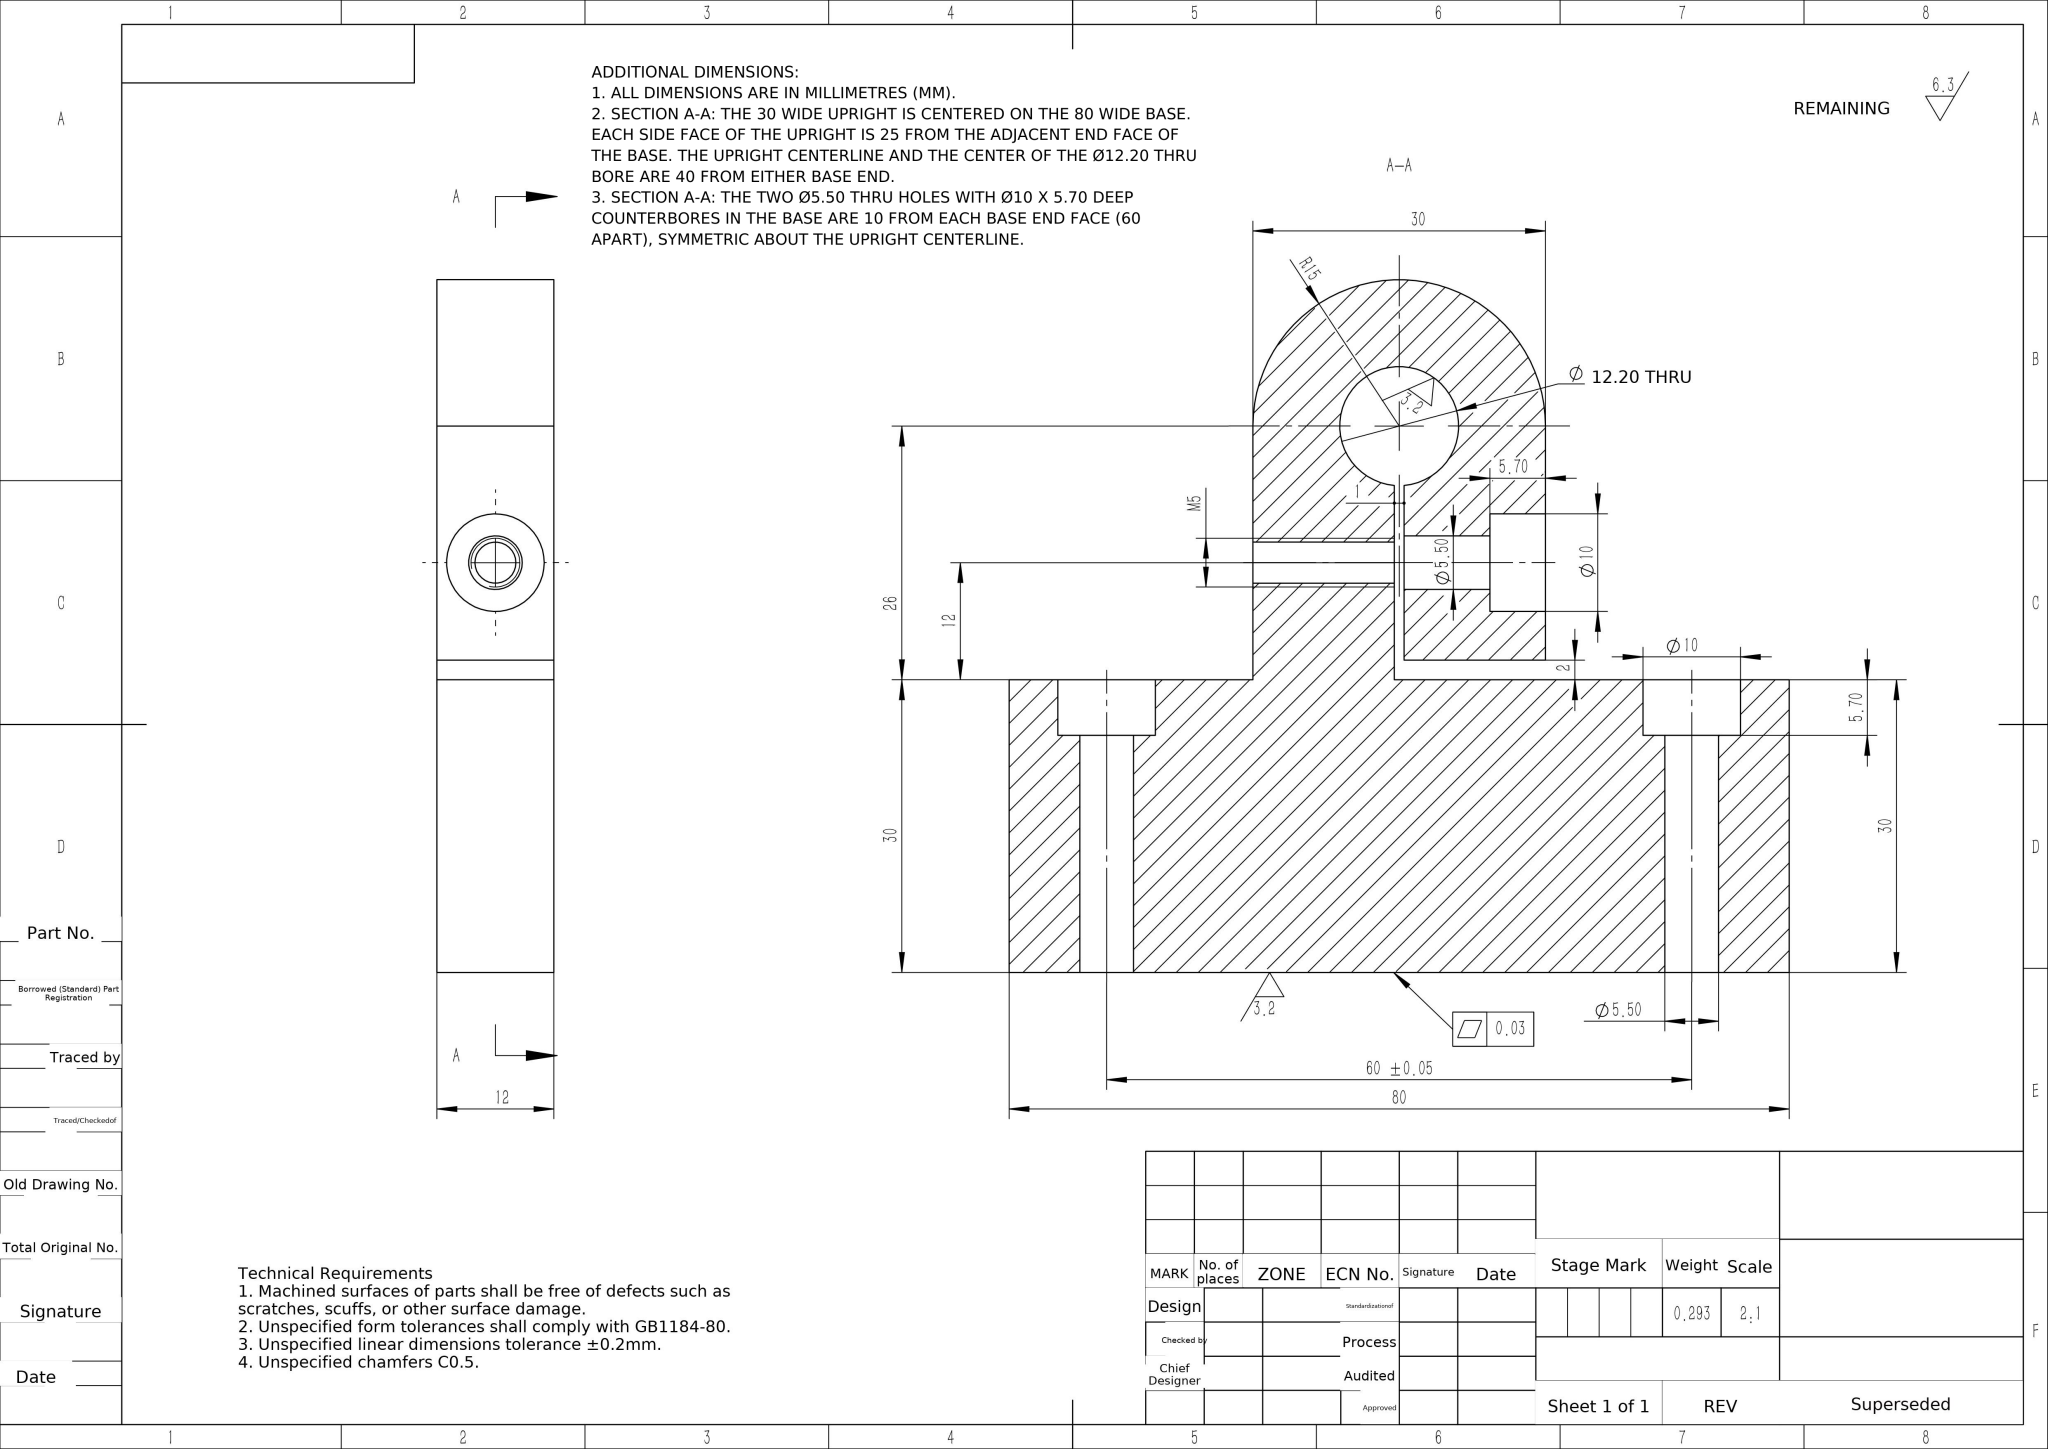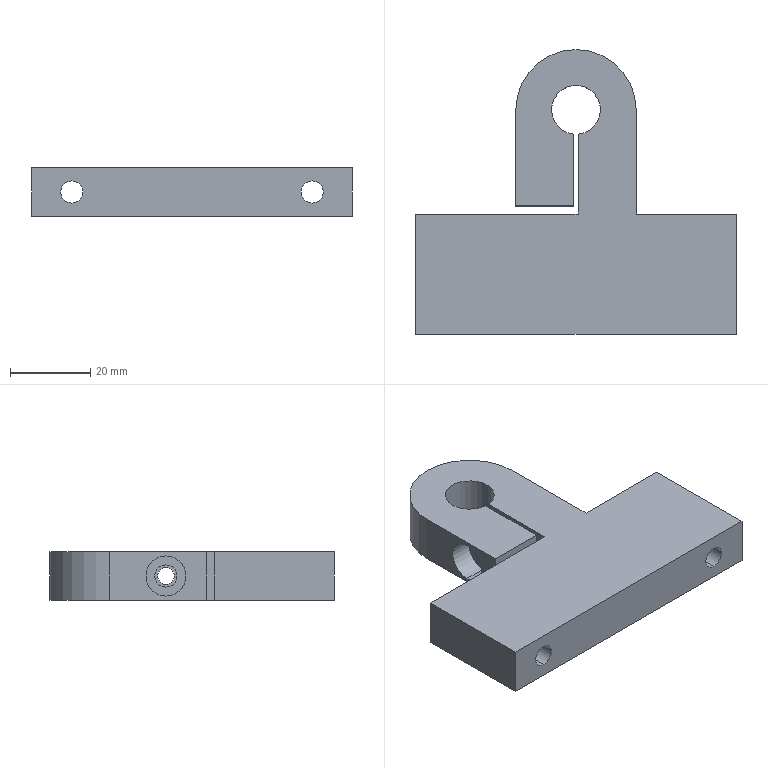Part | NX | mm | T-Shaped Dual-Bore Bracket | 1 solid | 33 faces | box 80 x 71 x 12 mm | volume 37504 mm3 | cylinder 18 | plane 15 | commonest cylinder face diameters 10 x6 5.5 x6 12.2 x3 4.2 x2 30 x1